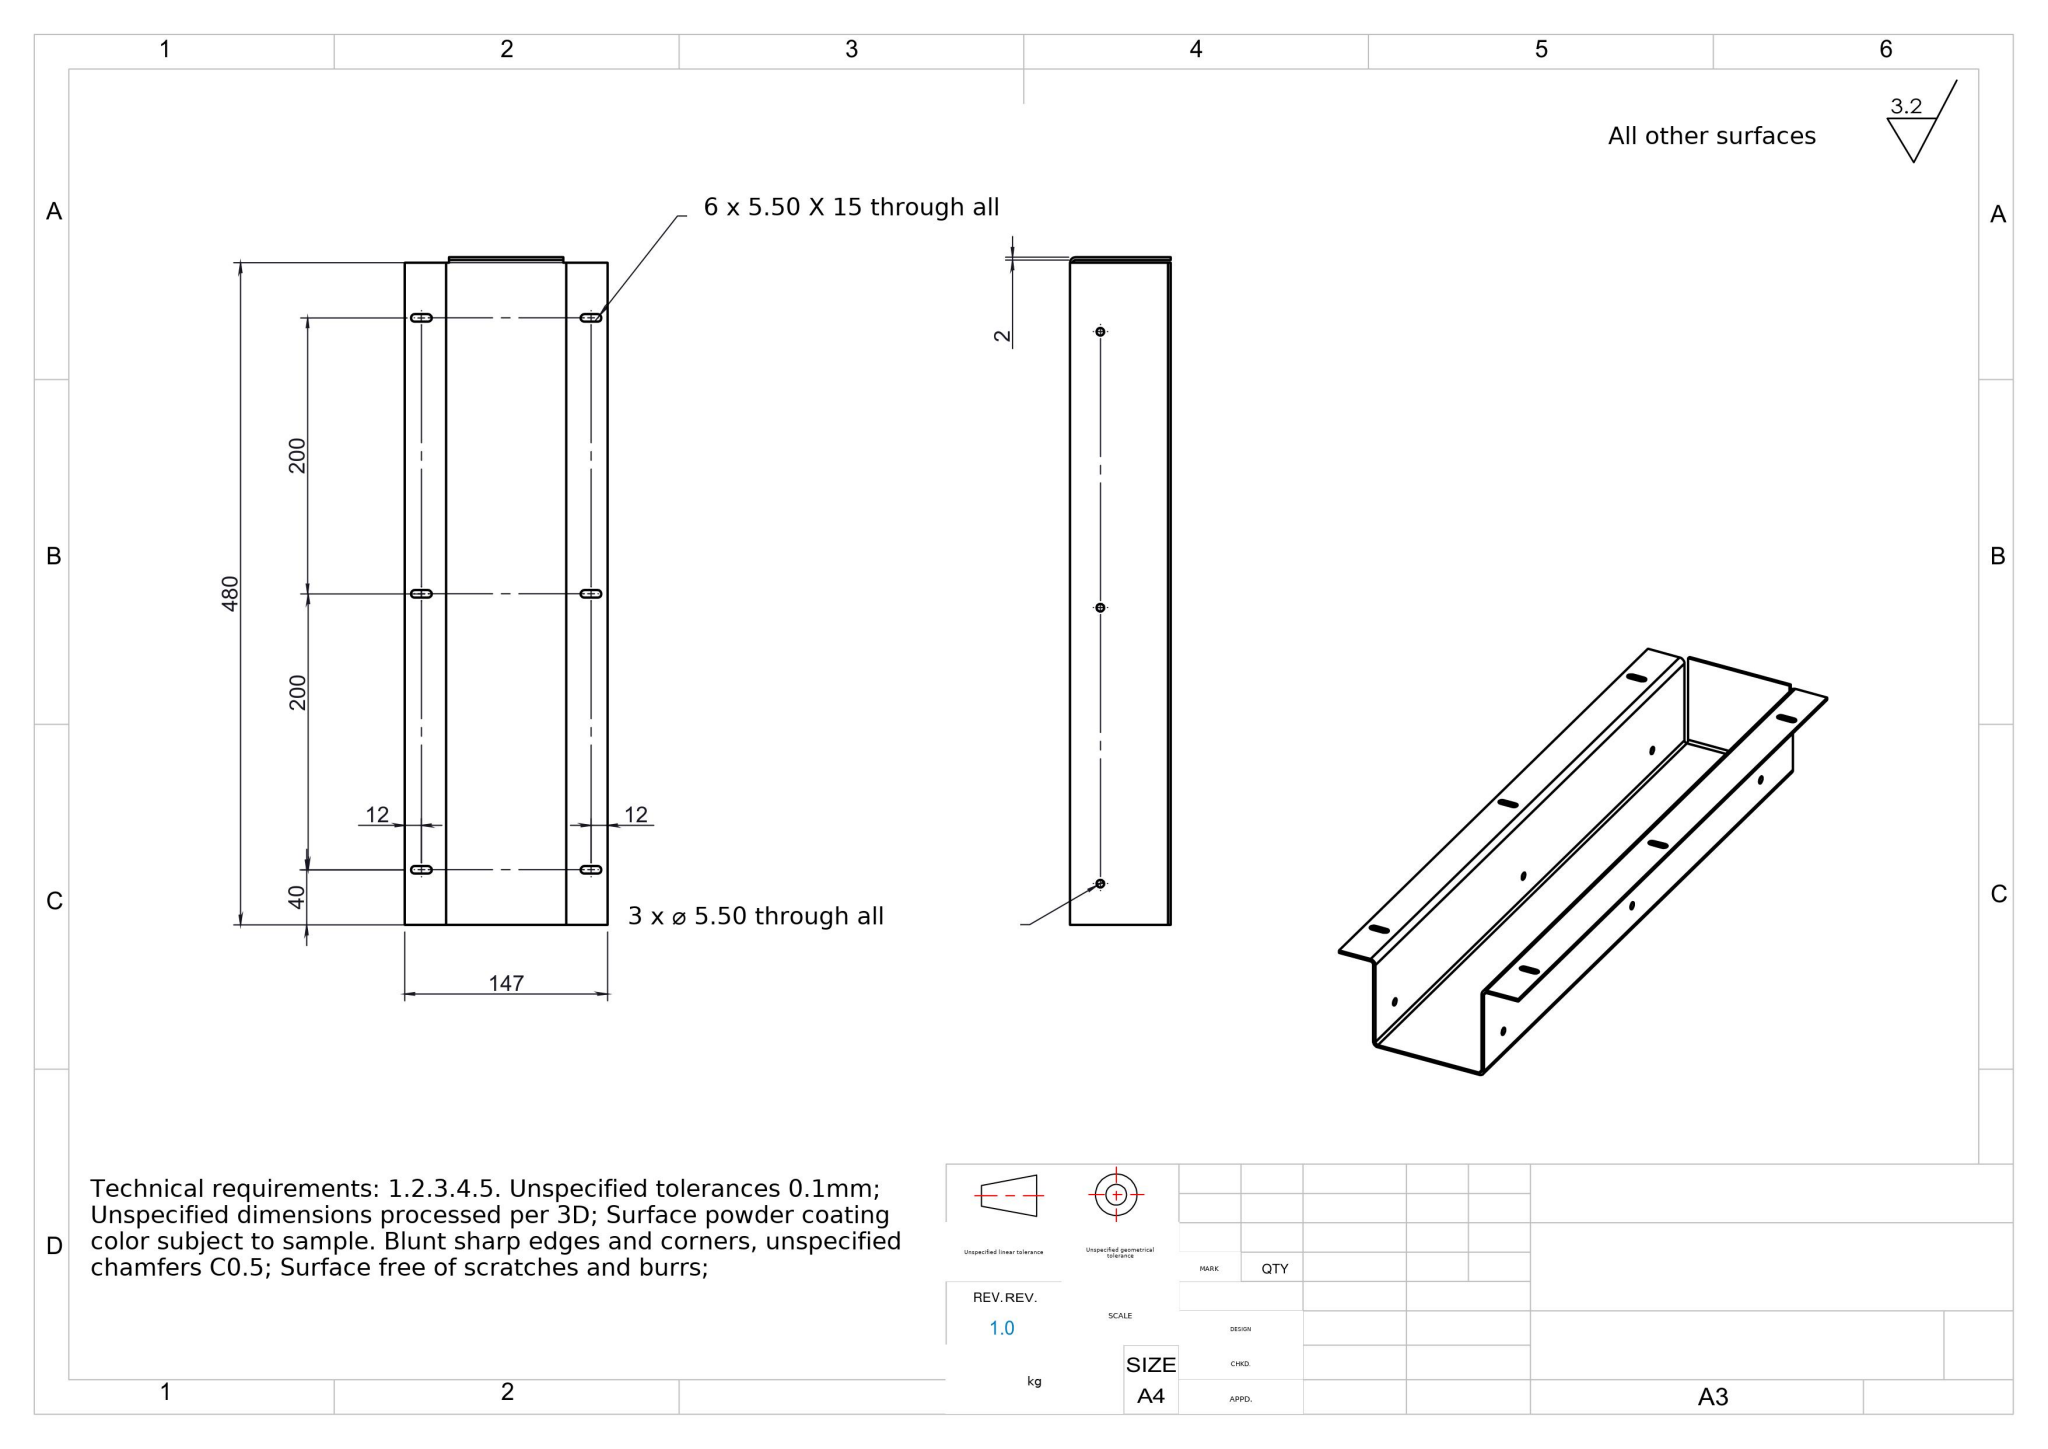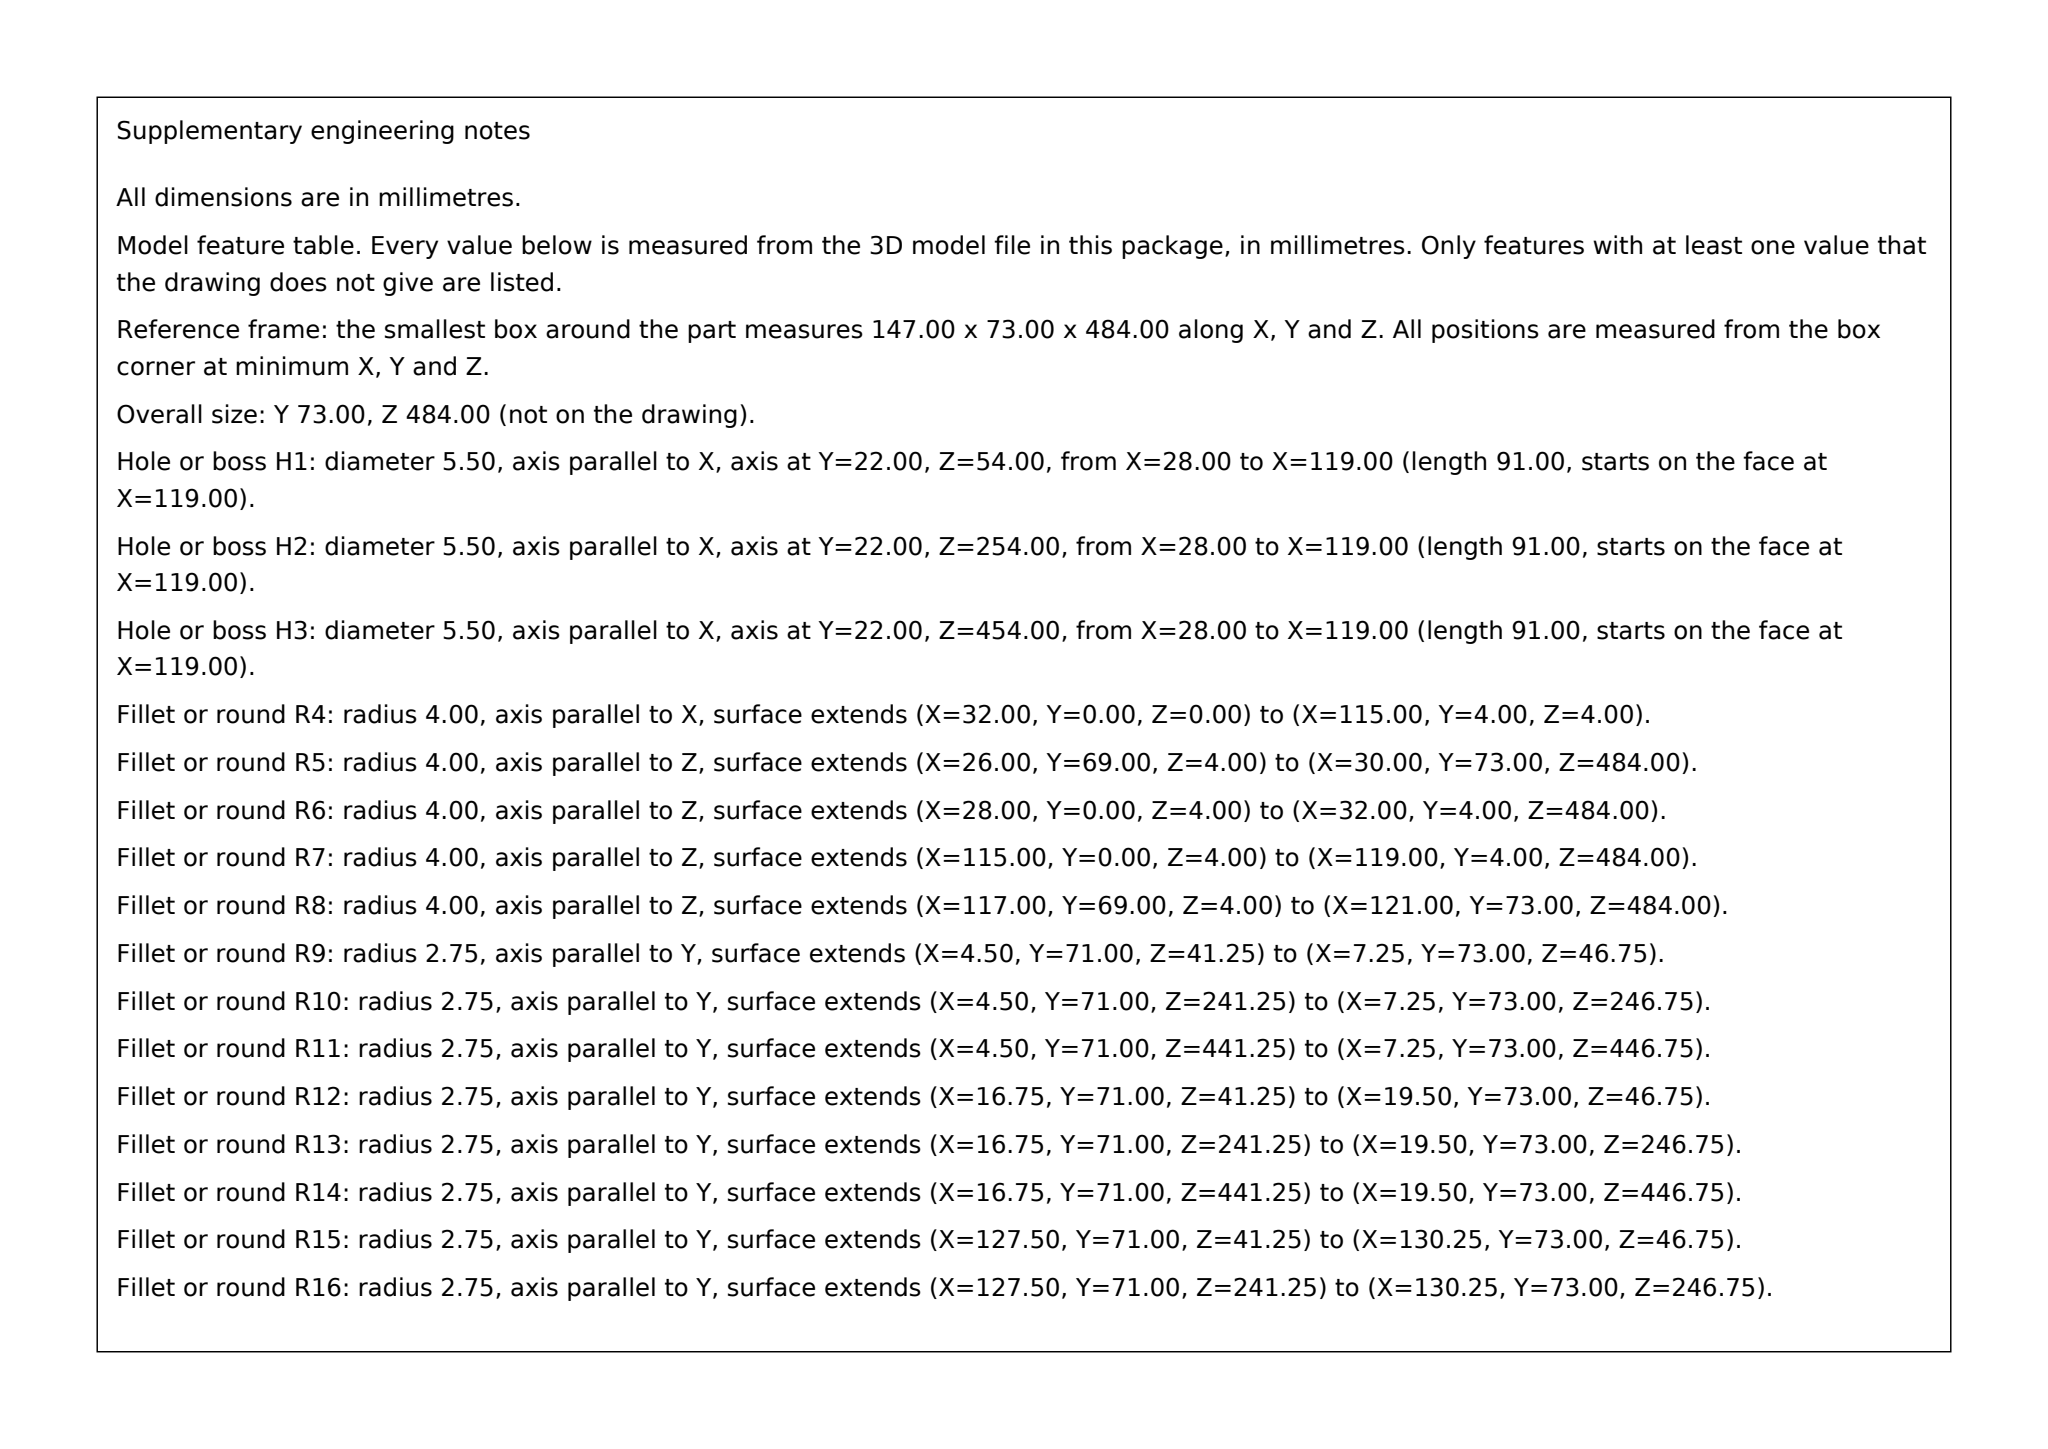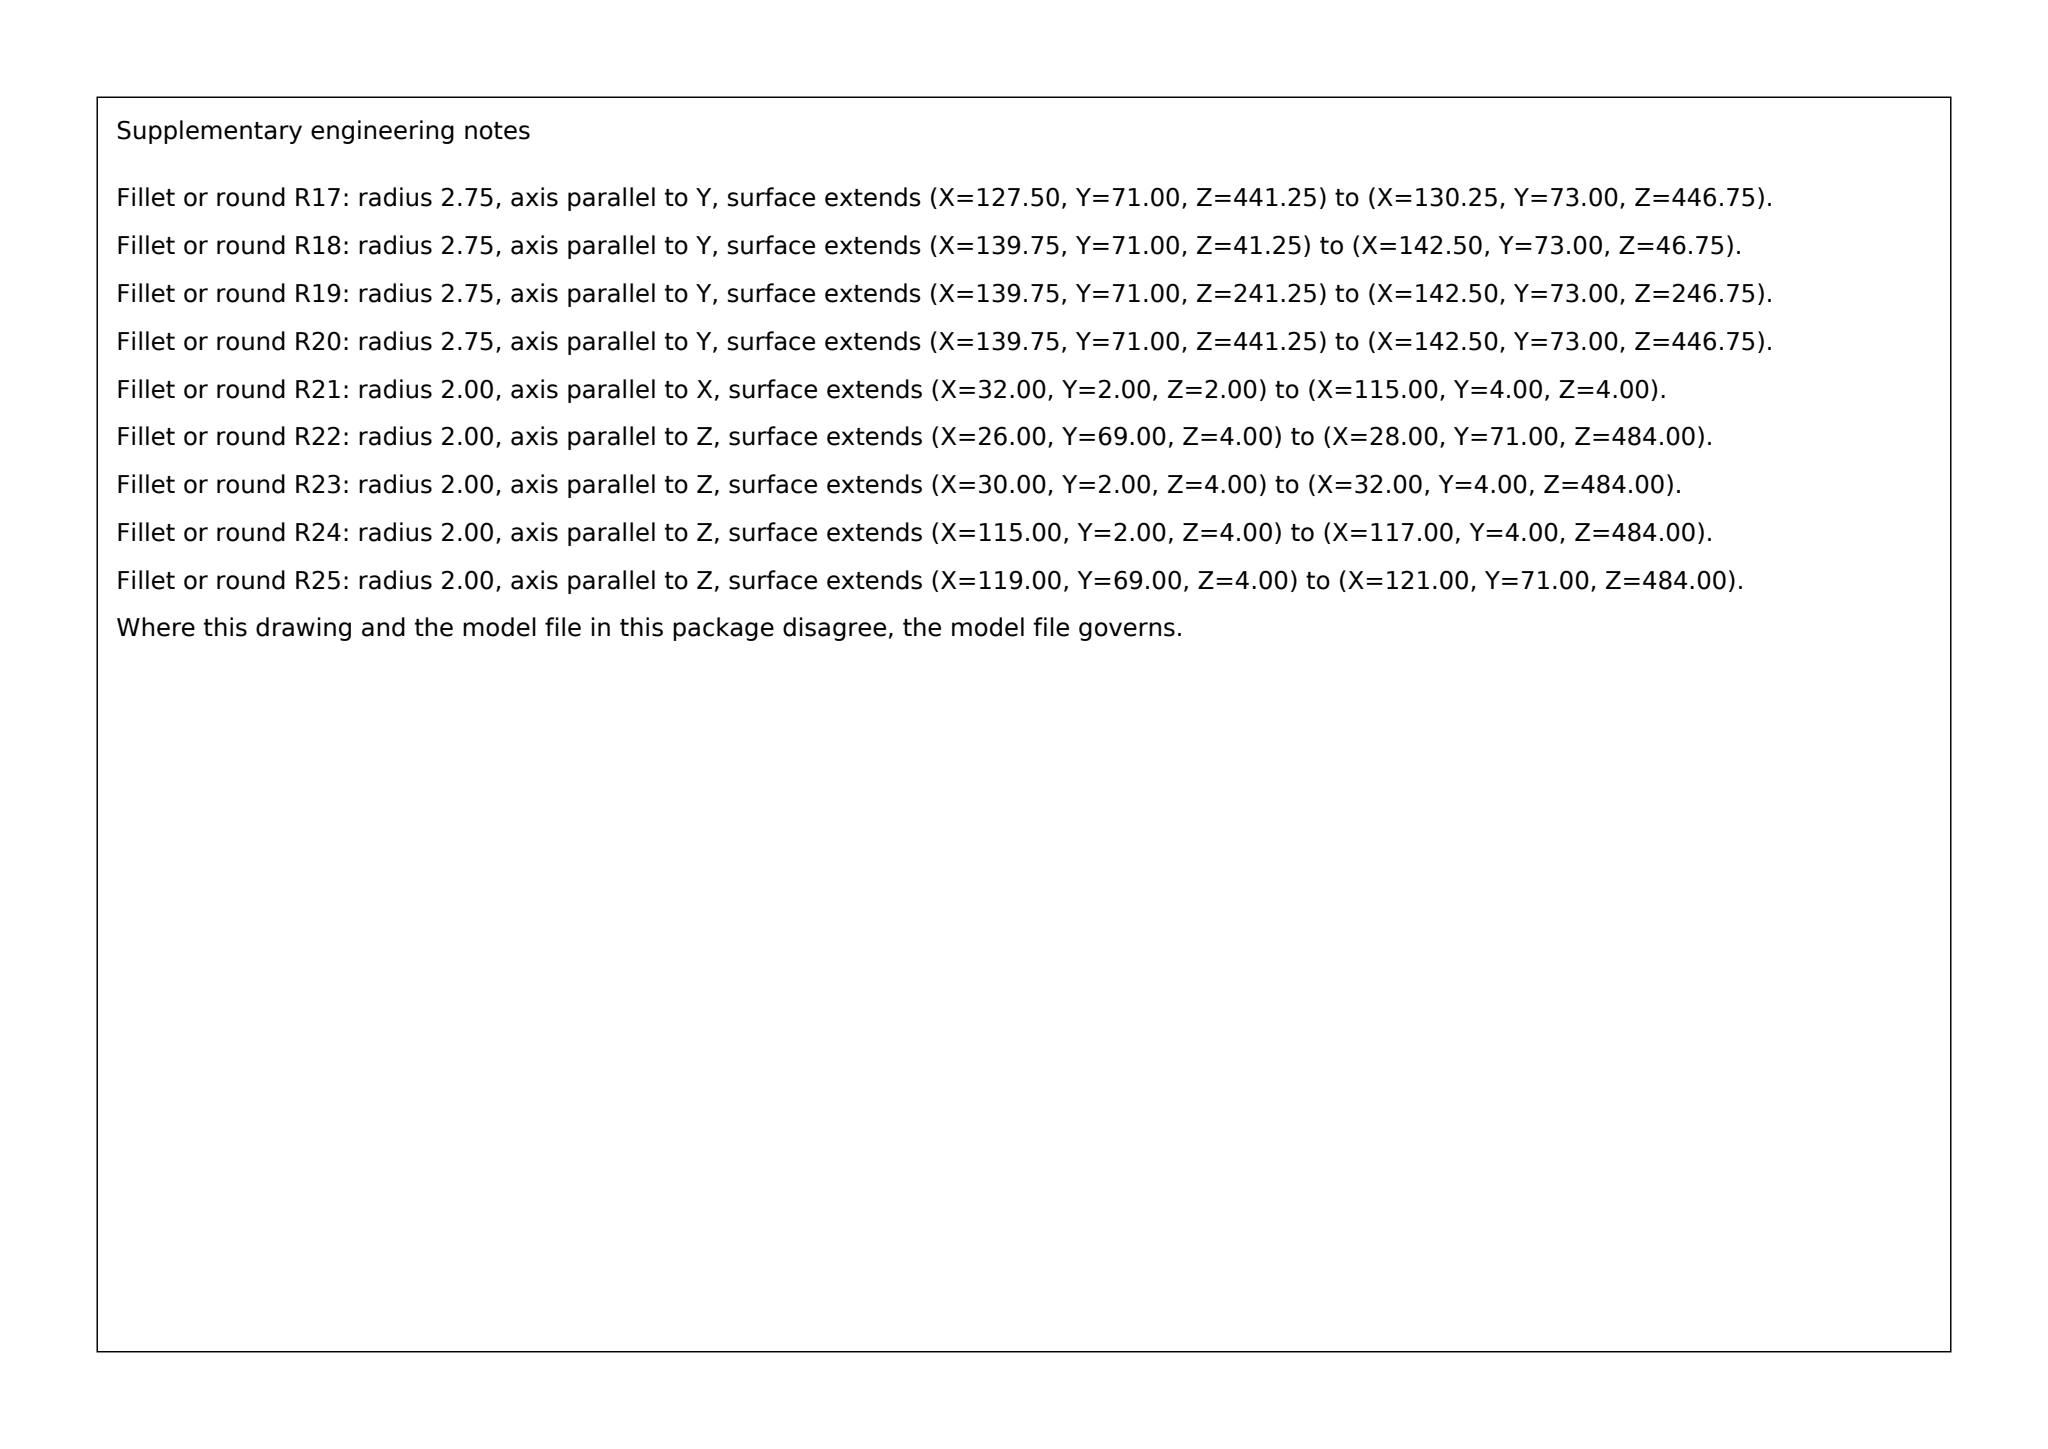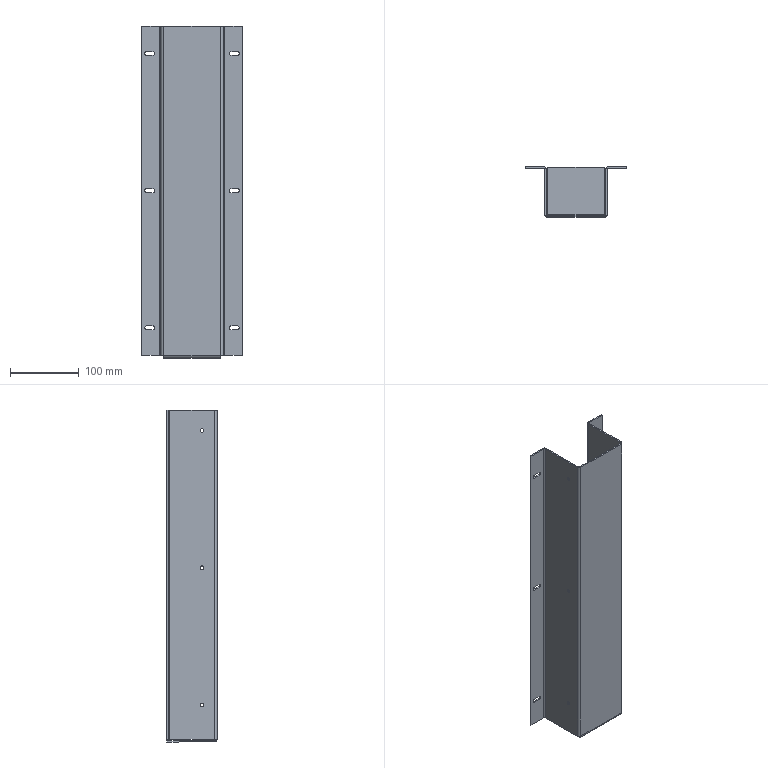Part | SolidWorks | mm | 1 solid | 82 faces | box 147 x 73 x 484 mm | volume 283535 mm3 | plane 48 | cylinder 34 | commonest cylinder face diameters 5.5 x24 8 x5 4 x5